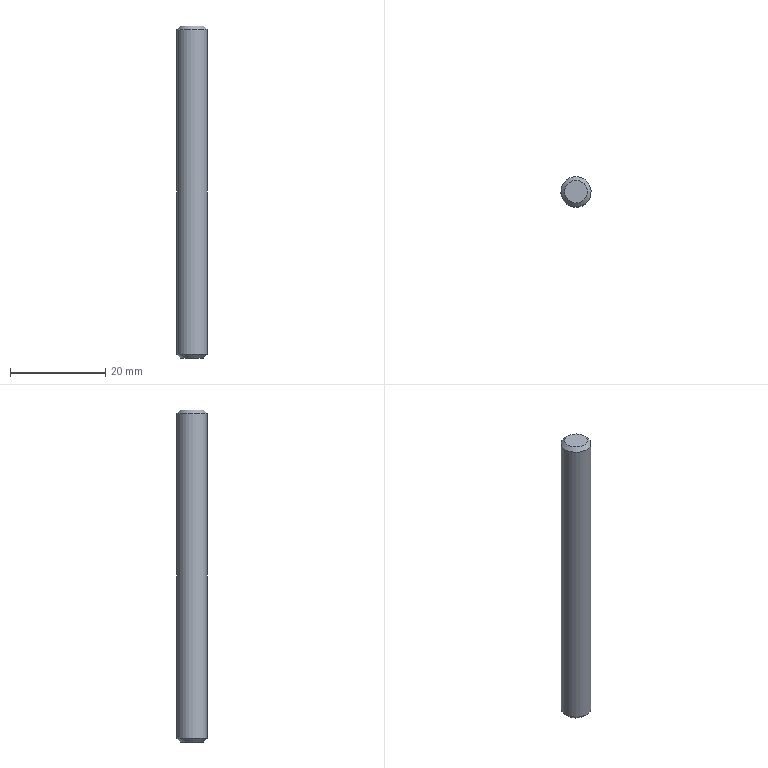Component | NX | MANIVELA | 1 solid | 5 faces | box 6.35 x 6.35 x 69.85 mm | volume 2201 mm3 | plane 2 | cone 2 | cylinder 1 | commonest cylinder face diameters 6.35 x1
STEP:
#1=CARTESIAN_POINT('',(0.,0.,0.));
#2=DIRECTION('',(0.,0.,1.));
#3=DIRECTION('',(1.,0.,0.));
#4=AXIS2_PLACEMENT_3D('',#1,#2,#3);
#5=CARTESIAN_POINT('',(139.022,80.588,41.118));
#6=VERTEX_POINT('',#5);
#7=CARTESIAN_POINT('',(139.574,77.461,41.118));
#8=DIRECTION('',(0.,0.,-1.));
#9=DIRECTION('',(-0.1736,0.9848,0.));
#10=AXIS2_PLACEMENT_3D('',#7,#8,#9);
#11=CIRCLE('',#10,3.175);
#12=CARTESIAN_POINT('',(139.574,77.461,41.912));
#13=DIRECTION('',(0.,0.,-1.));
#14=DIRECTION('',(-0.1736,0.9848,0.));
#15=AXIS2_PLACEMENT_3D('',#12,#13,#14);
#16=CYLINDRICAL_SURFACE('',#15,3.175);
#17=CARTESIAN_POINT('',(0.,0.7937));
#18=DIRECTION('',(1.,0.));
#19=VECTOR('',#18,1.);
#20=LINE('',#17,#19);
#21=(GEOMETRIC_REPRESENTATION_CONTEXT(2)PARAMETRIC_REPRESENTATION_CONTEXT()REPRESENTATION_CONTEXT('',''));
#22=DEFINITIONAL_REPRESENTATION('',(#20),#21);
#23=PCURVE('',#16,#22);
#24=CARTESIAN_POINT('',(139.574,77.461,41.118));
#25=DIRECTION('',(0.,0.,-1.));
#26=DIRECTION('',(-0.1736,0.9848,0.));
#27=AXIS2_PLACEMENT_3D('',#24,#25,#26);
#28=CONICAL_SURFACE('',#27,3.175,0.7854);
#29=CARTESIAN_POINT('',(0.,0.));
#30=DIRECTION('',(1.,0.));
#31=VECTOR('',#30,1.);
#32=LINE('',#29,#31);
#33=(GEOMETRIC_REPRESENTATION_CONTEXT(2)PARAMETRIC_REPRESENTATION_CONTEXT()REPRESENTATION_CONTEXT('',''));
#34=DEFINITIONAL_REPRESENTATION('',(#32),#33);
#35=PCURVE('',#28,#34);
#36=SURFACE_CURVE('',#11,(#23,#35),.PCURVE_S1.);
#37=EDGE_CURVE('',#6,#6,#36,.T.);
#38=ORIENTED_EDGE('',*,*,#37,.T.);
#39=CARTESIAN_POINT('',(139.022,80.588,-27.144));
#40=VERTEX_POINT('',#39);
#41=CARTESIAN_POINT('',(139.022,80.588,41.118));
#42=CARTESIAN_POINT('',(139.022,80.588,-27.144));
#43=B_SPLINE_CURVE_WITH_KNOTS('',1,(#41,#42),.UNSPECIFIED.,.F.,.F.,(2,2),(0.7937,69.056),.PIECEWISE_BEZIER_KNOTS.);
#44=CARTESIAN_POINT('',(6.283,0.));
#45=DIRECTION('',(0.,1.));
#46=VECTOR('',#45,1.);
#47=LINE('',#44,#46);
#48=(GEOMETRIC_REPRESENTATION_CONTEXT(2)PARAMETRIC_REPRESENTATION_CONTEXT()REPRESENTATION_CONTEXT('',''));
#49=DEFINITIONAL_REPRESENTATION('',(#47),#48);
#50=PCURVE('',#16,#49);
#51=CARTESIAN_POINT('',(0.,0.));
#52=DIRECTION('',(0.,1.));
#53=VECTOR('',#52,1.);
#54=LINE('',#51,#53);
#55=(GEOMETRIC_REPRESENTATION_CONTEXT(2)PARAMETRIC_REPRESENTATION_CONTEXT()REPRESENTATION_CONTEXT('',''));
#56=DEFINITIONAL_REPRESENTATION('',(#54),#55);
#57=PCURVE('',#16,#56);
#58=SEAM_CURVE('',#43,(#50,#57),.PCURVE_S1.);
#59=EDGE_CURVE('',#6,#40,#58,.T.);
#60=ORIENTED_EDGE('',*,*,#59,.T.);
#61=CARTESIAN_POINT('',(139.574,77.461,-27.144));
#62=DIRECTION('',(0.,0.,1.));
#63=DIRECTION('',(-0.1736,0.9848,0.));
#64=AXIS2_PLACEMENT_3D('',#61,#62,#63);
#65=CIRCLE('',#64,3.175);
#66=CARTESIAN_POINT('',(6.283,69.056));
#67=DIRECTION('',(-1.,0.));
#68=VECTOR('',#67,1.);
#69=LINE('',#66,#68);
#70=(GEOMETRIC_REPRESENTATION_CONTEXT(2)PARAMETRIC_REPRESENTATION_CONTEXT()REPRESENTATION_CONTEXT('',''));
#71=DEFINITIONAL_REPRESENTATION('',(#69),#70);
#72=PCURVE('',#16,#71);
#73=CARTESIAN_POINT('',(139.574,77.461,-27.938));
#74=DIRECTION('',(0.,0.,1.));
#75=DIRECTION('',(0.1736,-0.9848,0.));
#76=AXIS2_PLACEMENT_3D('',#73,#74,#75);
#77=CONICAL_SURFACE('',#76,2.381,0.7854);
#78=CARTESIAN_POINT('',(3.142,0.7938));
#79=DIRECTION('',(1.,0.));
#80=VECTOR('',#79,1.);
#81=LINE('',#78,#80);
#82=(GEOMETRIC_REPRESENTATION_CONTEXT(2)PARAMETRIC_REPRESENTATION_CONTEXT()REPRESENTATION_CONTEXT('',''));
#83=DEFINITIONAL_REPRESENTATION('',(#81),#82);
#84=PCURVE('',#77,#83);
#85=SURFACE_CURVE('',#65,(#72,#84),.PCURVE_S1.);
#86=EDGE_CURVE('',#40,#40,#85,.T.);
#87=ORIENTED_EDGE('',*,*,#86,.T.);
#88=ORIENTED_EDGE('',*,*,#59,.F.);
#89=EDGE_LOOP('',(#38,#60,#87,#88));
#90=FACE_BOUND('',#89,.T.);
#91=ADVANCED_FACE('',(#90),#16,.T.);
#92=CARTESIAN_POINT('',(139.16,79.806,41.912));
#93=VERTEX_POINT('',#92);
#94=CARTESIAN_POINT('',(139.574,77.461,41.912));
#95=DIRECTION('',(0.,0.,1.));
#96=DIRECTION('',(-0.1736,0.9848,0.));
#97=AXIS2_PLACEMENT_3D('',#94,#95,#96);
#98=CIRCLE('',#97,2.381);
#99=CARTESIAN_POINT('',(139.574,77.461,41.912));
#100=DIRECTION('',(0.,0.,-1.));
#101=DIRECTION('',(-0.1736,0.9848,0.));
#102=AXIS2_PLACEMENT_3D('',#99,#100,#101);
#103=PLANE('',#102);
#104=CARTESIAN_POINT('',(2.381,0.));
#105=CARTESIAN_POINT('',(2.381,-4.124));
#106=CARTESIAN_POINT('',(-1.191,-2.062));
#107=CARTESIAN_POINT('',(-4.763,-0.));
#108=CARTESIAN_POINT('',(-1.191,2.062));
#109=CARTESIAN_POINT('',(2.381,4.124));
#110=CARTESIAN_POINT('',(2.381,0.));
#111=(BOUNDED_CURVE()B_SPLINE_CURVE(2,(#104,#105,#106,#107,#108,#109,#110),.UNSPECIFIED.,.T.,.F.)B_SPLINE_CURVE_WITH_KNOTS((1,2,2,2,2,1),(-2.094,0.,2.094,4.189,6.283,8.378),.UNSPECIFIED.)CURVE()GEOMETRIC_REPRESENTATION_ITEM()RATIONAL_B_SPLINE_CURVE((1.,0.5,1.,0.5,1.,0.5,1.))REPRESENTATION_ITEM(''));
#112=(GEOMETRIC_REPRESENTATION_CONTEXT(2)PARAMETRIC_REPRESENTATION_CONTEXT()REPRESENTATION_CONTEXT('',''));
#113=DEFINITIONAL_REPRESENTATION('',(#111),#112);
#114=PCURVE('',#103,#113);
#115=CARTESIAN_POINT('',(6.283,-0.7938));
#116=DIRECTION('',(-1.,0.));
#117=VECTOR('',#116,1.);
#118=LINE('',#115,#117);
#119=(GEOMETRIC_REPRESENTATION_CONTEXT(2)PARAMETRIC_REPRESENTATION_CONTEXT()REPRESENTATION_CONTEXT('',''));
#120=DEFINITIONAL_REPRESENTATION('',(#118),#119);
#121=PCURVE('',#28,#120);
#122=SURFACE_CURVE('',#98,(#114,#121),.PCURVE_S1.);
#123=EDGE_CURVE('',#93,#93,#122,.T.);
#124=ORIENTED_EDGE('',*,*,#123,.T.);
#125=EDGE_LOOP('',(#124));
#126=FACE_BOUND('',#125,.T.);
#127=ADVANCED_FACE('',(#126),#103,.F.);
#128=CARTESIAN_POINT('',(139.16,79.806,-27.938));
#129=VERTEX_POINT('',#128);
#130=CARTESIAN_POINT('',(139.574,77.461,-27.938));
#131=DIRECTION('',(0.,0.,-1.));
#132=DIRECTION('',(-0.1736,0.9848,0.));
#133=AXIS2_PLACEMENT_3D('',#130,#131,#132);
#134=CIRCLE('',#133,2.381);
#135=CARTESIAN_POINT('',(139.574,77.461,-27.938));
#136=DIRECTION('',(0.,0.,-1.));
#137=DIRECTION('',(-0.1736,0.9848,0.));
#138=AXIS2_PLACEMENT_3D('',#135,#136,#137);
#139=PLANE('',#138);
#140=CARTESIAN_POINT('',(0.,0.));
#141=DIRECTION('',(1.,0.));
#142=AXIS2_PLACEMENT_2D('',#140,#141);
#143=CIRCLE('',#142,2.381);
#144=(GEOMETRIC_REPRESENTATION_CONTEXT(2)PARAMETRIC_REPRESENTATION_CONTEXT()REPRESENTATION_CONTEXT('',''));
#145=DEFINITIONAL_REPRESENTATION('',(#143),#144);
#146=PCURVE('',#139,#145);
#147=CARTESIAN_POINT('',(9.425,0.));
#148=DIRECTION('',(-1.,0.));
#149=VECTOR('',#148,1.);
#150=LINE('',#147,#149);
#151=(GEOMETRIC_REPRESENTATION_CONTEXT(2)PARAMETRIC_REPRESENTATION_CONTEXT()REPRESENTATION_CONTEXT('',''));
#152=DEFINITIONAL_REPRESENTATION('',(#150),#151);
#153=PCURVE('',#77,#152);
#154=SURFACE_CURVE('',#134,(#146,#153),.PCURVE_S1.);
#155=EDGE_CURVE('',#129,#129,#154,.T.);
#156=ORIENTED_EDGE('',*,*,#155,.T.);
#157=EDGE_LOOP('',(#156));
#158=FACE_BOUND('',#157,.T.);
#159=ADVANCED_FACE('',(#158),#139,.T.);
#160=ORIENTED_EDGE('',*,*,#86,.F.);
#161=CARTESIAN_POINT('',(139.16,79.806,-27.938));
#162=CARTESIAN_POINT('',(139.022,80.588,-27.144));
#163=B_SPLINE_CURVE_WITH_KNOTS('',1,(#161,#162),.UNSPECIFIED.,.F.,.F.,(2,2),(0.,1.123),.PIECEWISE_BEZIER_KNOTS.);
#164=CARTESIAN_POINT('',(3.142,0.));
#165=DIRECTION('',(0.,1.));
#166=VECTOR('',#165,1.);
#167=LINE('',#164,#166);
#168=(GEOMETRIC_REPRESENTATION_CONTEXT(2)PARAMETRIC_REPRESENTATION_CONTEXT()REPRESENTATION_CONTEXT('',''));
#169=DEFINITIONAL_REPRESENTATION('',(#167),#168);
#170=PCURVE('',#77,#169);
#171=CARTESIAN_POINT('',(9.425,0.));
#172=DIRECTION('',(0.,1.));
#173=VECTOR('',#172,1.);
#174=LINE('',#171,#173);
#175=(GEOMETRIC_REPRESENTATION_CONTEXT(2)PARAMETRIC_REPRESENTATION_CONTEXT()REPRESENTATION_CONTEXT('',''));
#176=DEFINITIONAL_REPRESENTATION('',(#174),#175);
#177=PCURVE('',#77,#176);
#178=SEAM_CURVE('',#163,(#170,#177),.PCURVE_S1.);
#179=EDGE_CURVE('',#129,#40,#178,.T.);
#180=ORIENTED_EDGE('',*,*,#179,.F.);
#181=ORIENTED_EDGE('',*,*,#155,.F.);
#182=ORIENTED_EDGE('',*,*,#179,.T.);
#183=EDGE_LOOP('',(#160,#180,#181,#182));
#184=FACE_BOUND('',#183,.T.);
#185=ADVANCED_FACE('',(#184),#77,.T.);
#186=ORIENTED_EDGE('',*,*,#123,.F.);
#187=CARTESIAN_POINT('',(139.16,79.806,41.912));
#188=CARTESIAN_POINT('',(139.022,80.588,41.118));
#189=B_SPLINE_CURVE_WITH_KNOTS('',1,(#187,#188),.UNSPECIFIED.,.F.,.F.,(2,2),(-1.123,0.),.PIECEWISE_BEZIER_KNOTS.);
#190=CARTESIAN_POINT('',(6.283,0.));
#191=DIRECTION('',(0.,1.));
#192=VECTOR('',#191,1.);
#193=LINE('',#190,#192);
#194=(GEOMETRIC_REPRESENTATION_CONTEXT(2)PARAMETRIC_REPRESENTATION_CONTEXT()REPRESENTATION_CONTEXT('',''));
#195=DEFINITIONAL_REPRESENTATION('',(#193),#194);
#196=PCURVE('',#28,#195);
#197=CARTESIAN_POINT('',(0.,0.));
#198=DIRECTION('',(0.,1.));
#199=VECTOR('',#198,1.);
#200=LINE('',#197,#199);
#201=(GEOMETRIC_REPRESENTATION_CONTEXT(2)PARAMETRIC_REPRESENTATION_CONTEXT()REPRESENTATION_CONTEXT('',''));
#202=DEFINITIONAL_REPRESENTATION('',(#200),#201);
#203=PCURVE('',#28,#202);
#204=SEAM_CURVE('',#189,(#196,#203),.PCURVE_S1.);
#205=EDGE_CURVE('',#93,#6,#204,.T.);
#206=ORIENTED_EDGE('',*,*,#205,.T.);
#207=ORIENTED_EDGE('',*,*,#37,.F.);
#208=ORIENTED_EDGE('',*,*,#205,.F.);
#209=EDGE_LOOP('',(#186,#206,#207,#208));
#210=FACE_BOUND('',#209,.T.);
#211=ADVANCED_FACE('',(#210),#28,.T.);
#212=CLOSED_SHELL('',(#91,#127,#159,#185,#211));
#213=MANIFOLD_SOLID_BREP('',#212);
#214=(LENGTH_UNIT()NAMED_UNIT(*)SI_UNIT(.MILLI.,.METRE.));
#215=UNCERTAINTY_MEASURE_WITH_UNIT(LENGTH_MEASURE(0.00001),#214,'','');
#216=(NAMED_UNIT(*)PLANE_ANGLE_UNIT()SI_UNIT($,.RADIAN.));
#217=(NAMED_UNIT(*)SI_UNIT($,.STERADIAN.)SOLID_ANGLE_UNIT());
#218=(GEOMETRIC_REPRESENTATION_CONTEXT(3)GLOBAL_UNCERTAINTY_ASSIGNED_CONTEXT((#215))GLOBAL_UNIT_ASSIGNED_CONTEXT((#214,#216,#217))REPRESENTATION_CONTEXT('',''));
#219=ADVANCED_BREP_SHAPE_REPRESENTATION('',(#4,#213),#218);